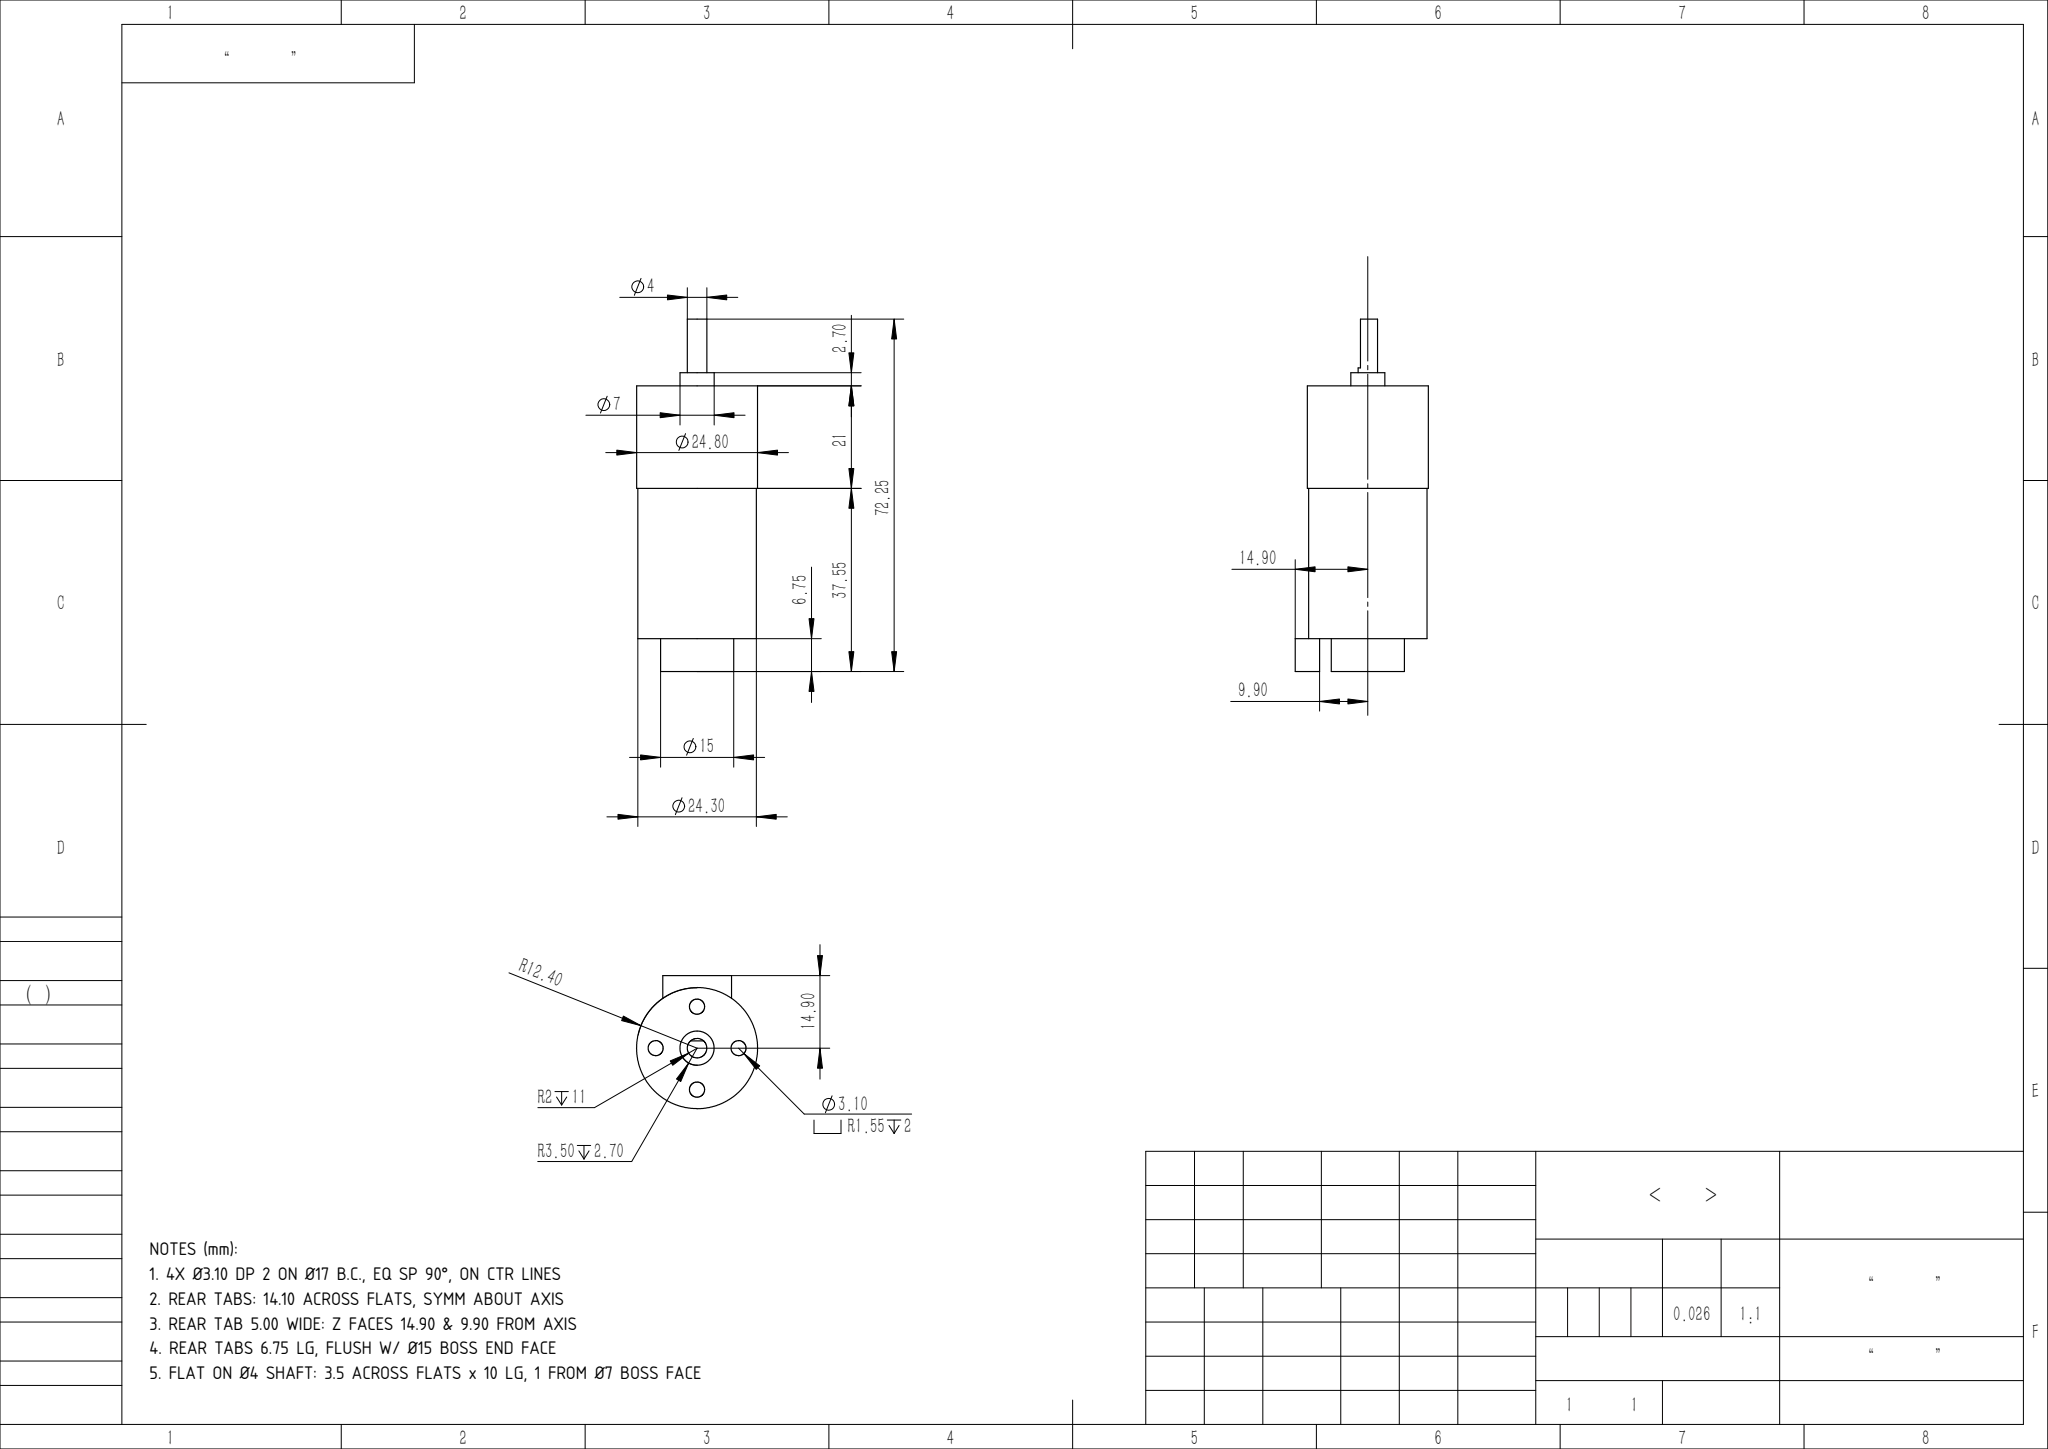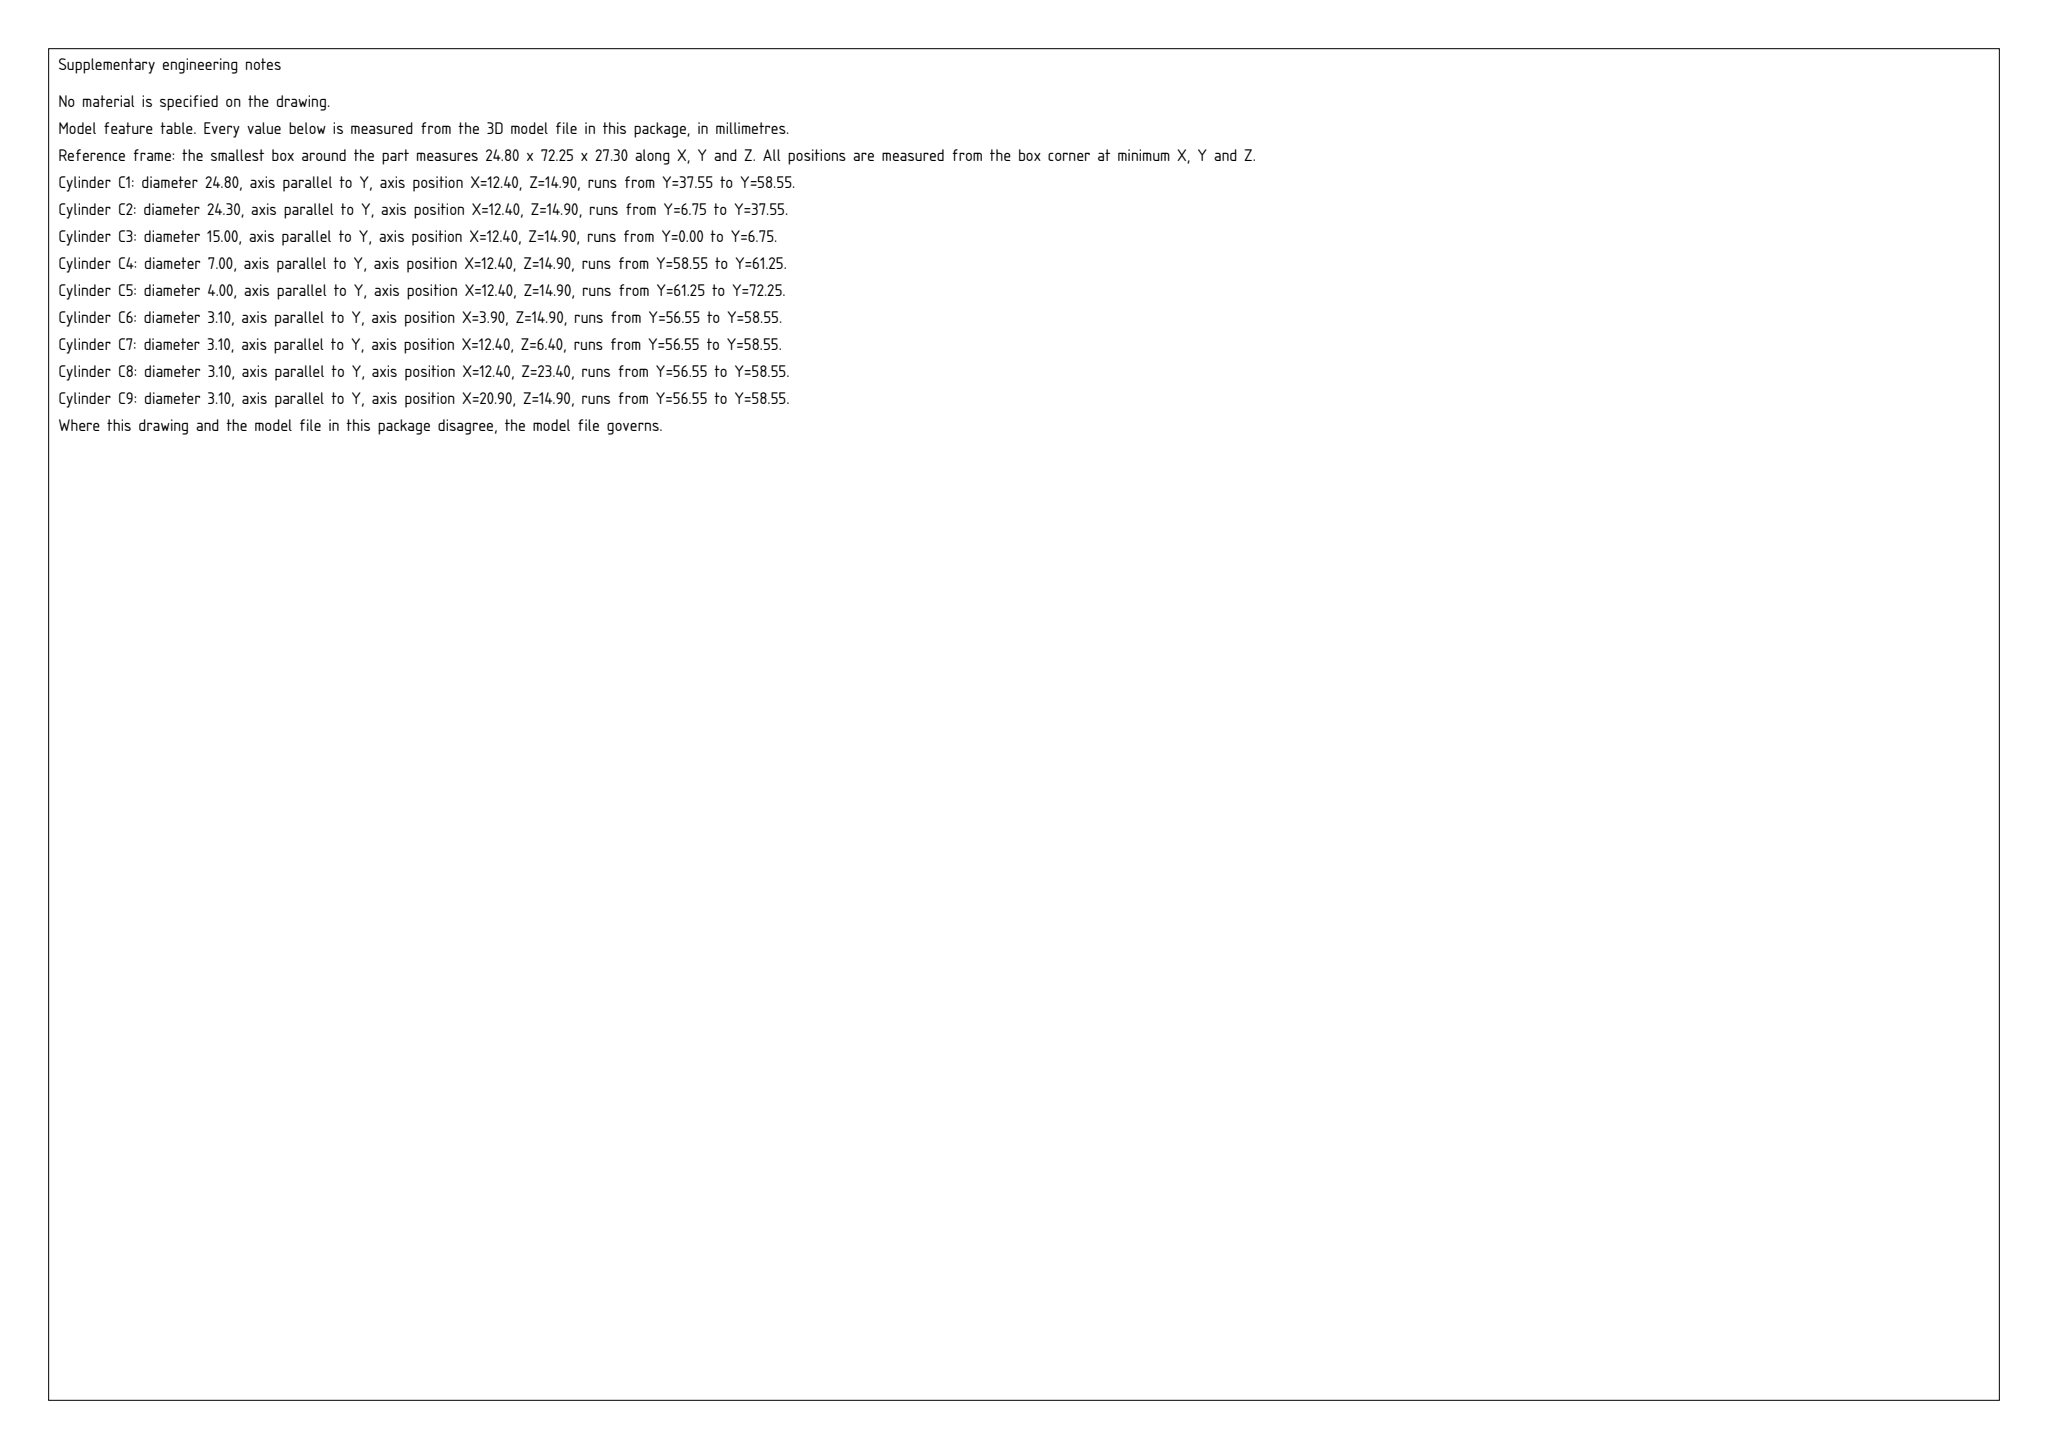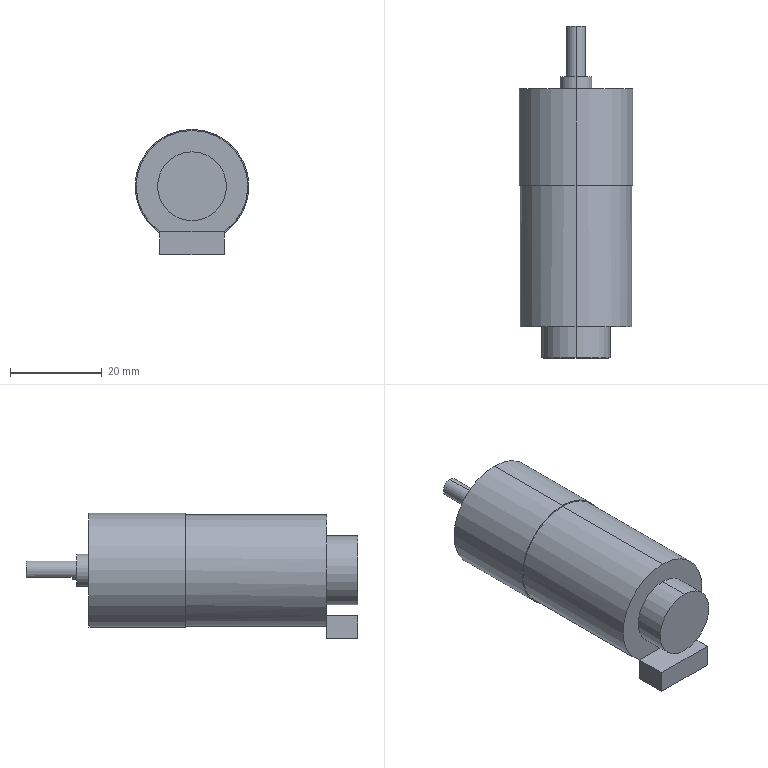Part | SolidWorks | mm | 1 solid | 36 faces | box 24.8 x 72.25 x 27.3 mm | volume 26270 mm3 | plane 18 | cylinder 18 | commonest cylinder face diameters 3.1 x8 15 x2 4 x2 7 x2 24.8 x2 24.3 x2
Drawing notes:
4X Ø3.10 DP 2 ON Ø17 B.C., EQ SP 90°, ON CTR LINES | from the solid: Ø3.1 y-holes at (3.9,14.9),(20.9,14.9),(12.4,6.4),(12.4,23.4); axis (12.4,14.9) => ±8.5 offsets = Ø17 B.C.; depth 2.0 from face y=58.55 to 56.55
REAR TABS: 14.10 ACROSS FLATS, SYMM ABOUT AXIS | from the solid: x-planes at 5.35 and 19.45; axis x=12.4 => 14.10 wide, ±7.05 symm
REAR TAB 5.00 WIDE: Z FACES 14.90 & 9.90 FROM AXIS | from the solid: z-planes 0.0 and 5.0; axis z=14.9 => 14.90 and 9.90, tab width 5.00
REAR TABS 6.75 LG, FLUSH W/ Ø15 BOSS END FACE | from the solid: y-planes 0.0 and 6.75 only in tab region; Ø15 boss length 6.75 from y=0 to 6.75
FLAT ON Ø4 SHAFT: 3.5 ACROSS FLATS x 10 LG, 1 FROM Ø7 BOSS FACE | from the solid: Ø4 shaft axis at (x12.4,z14.9), y61.25-72.25 (11 lg); planar face z=13.4 = 1.5 from axis => 3.5 across flats (0.5 deep); flat start plane y=62.25 to shaft end y=72.25 = 10 lg, 1.0 from Ø7 boss face y=61.25